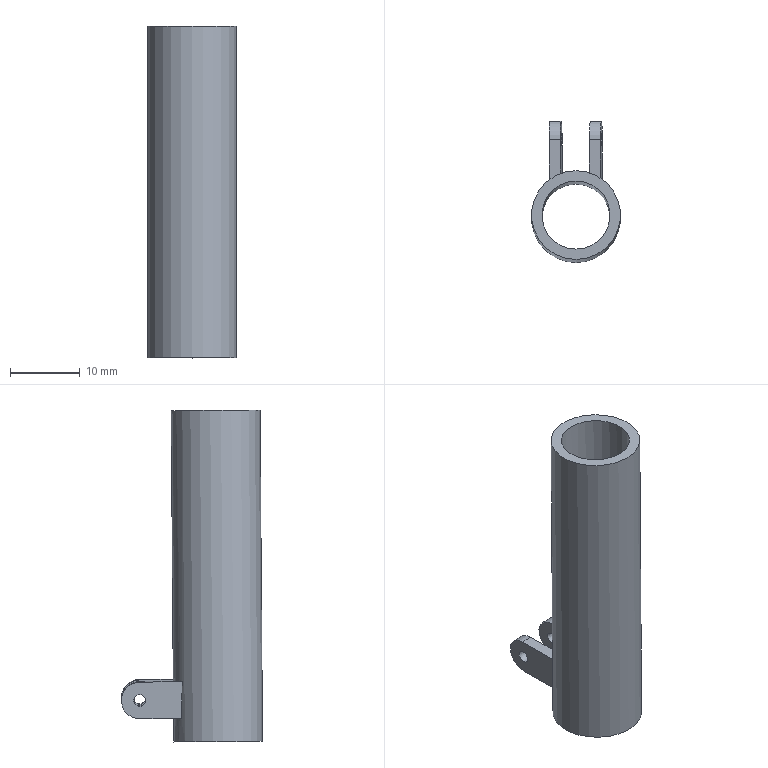Component | NX | CASING | 1 solid | 17 faces | volume 2644 mm3 | plane 11 | cylinder 6 | commonest cylinder face diameters 5.292 x2 1.7 x2 12.77 x1 9.78 x1